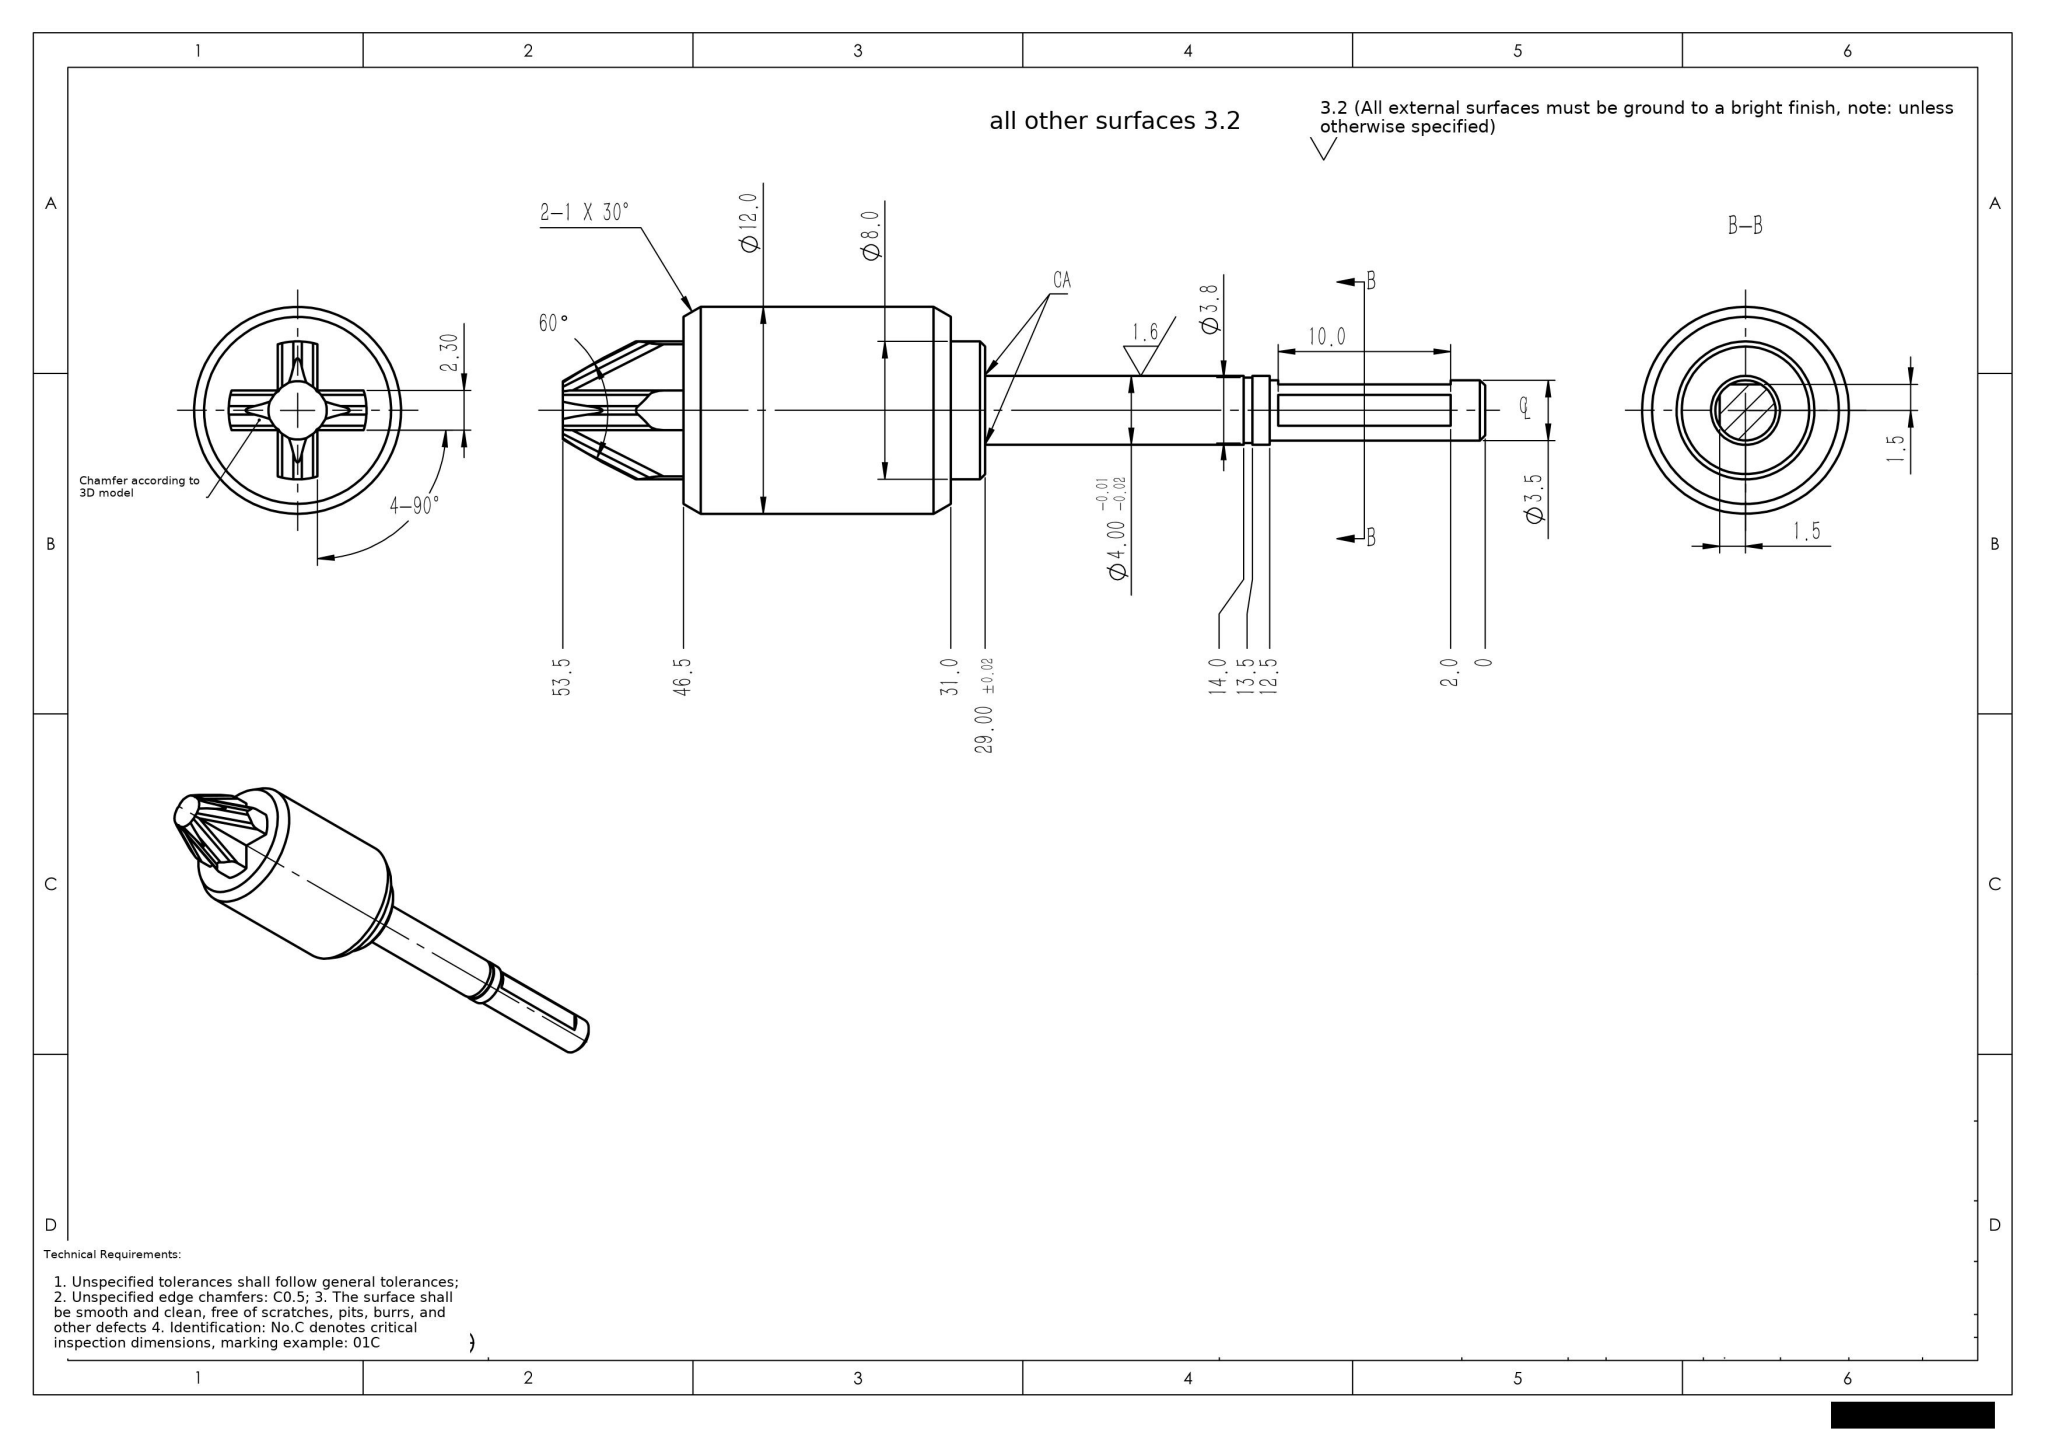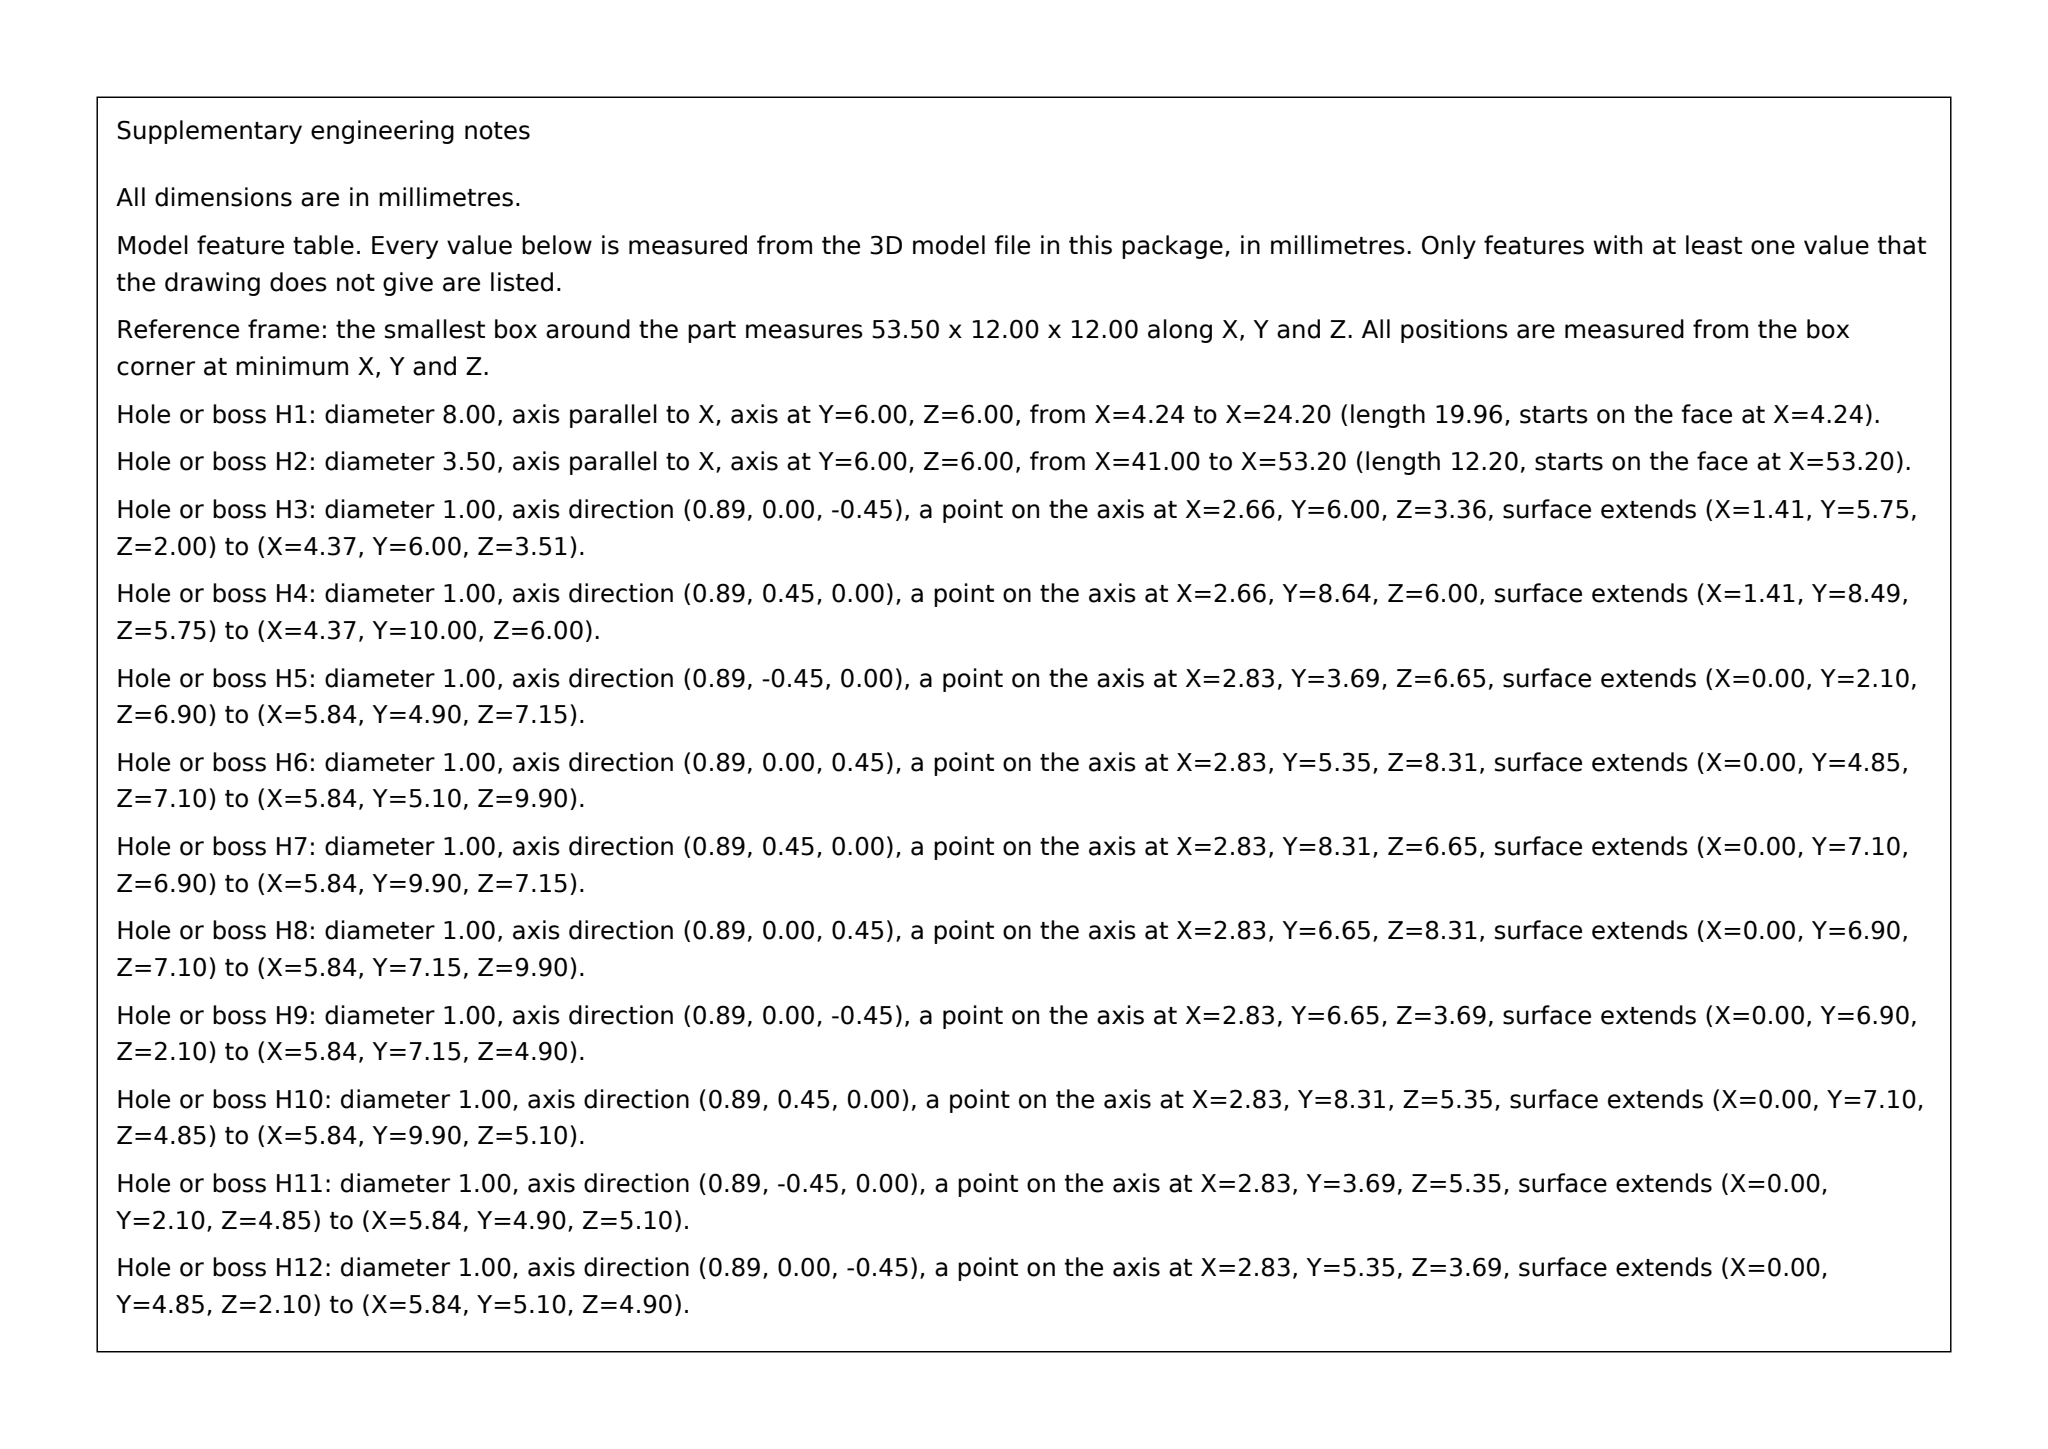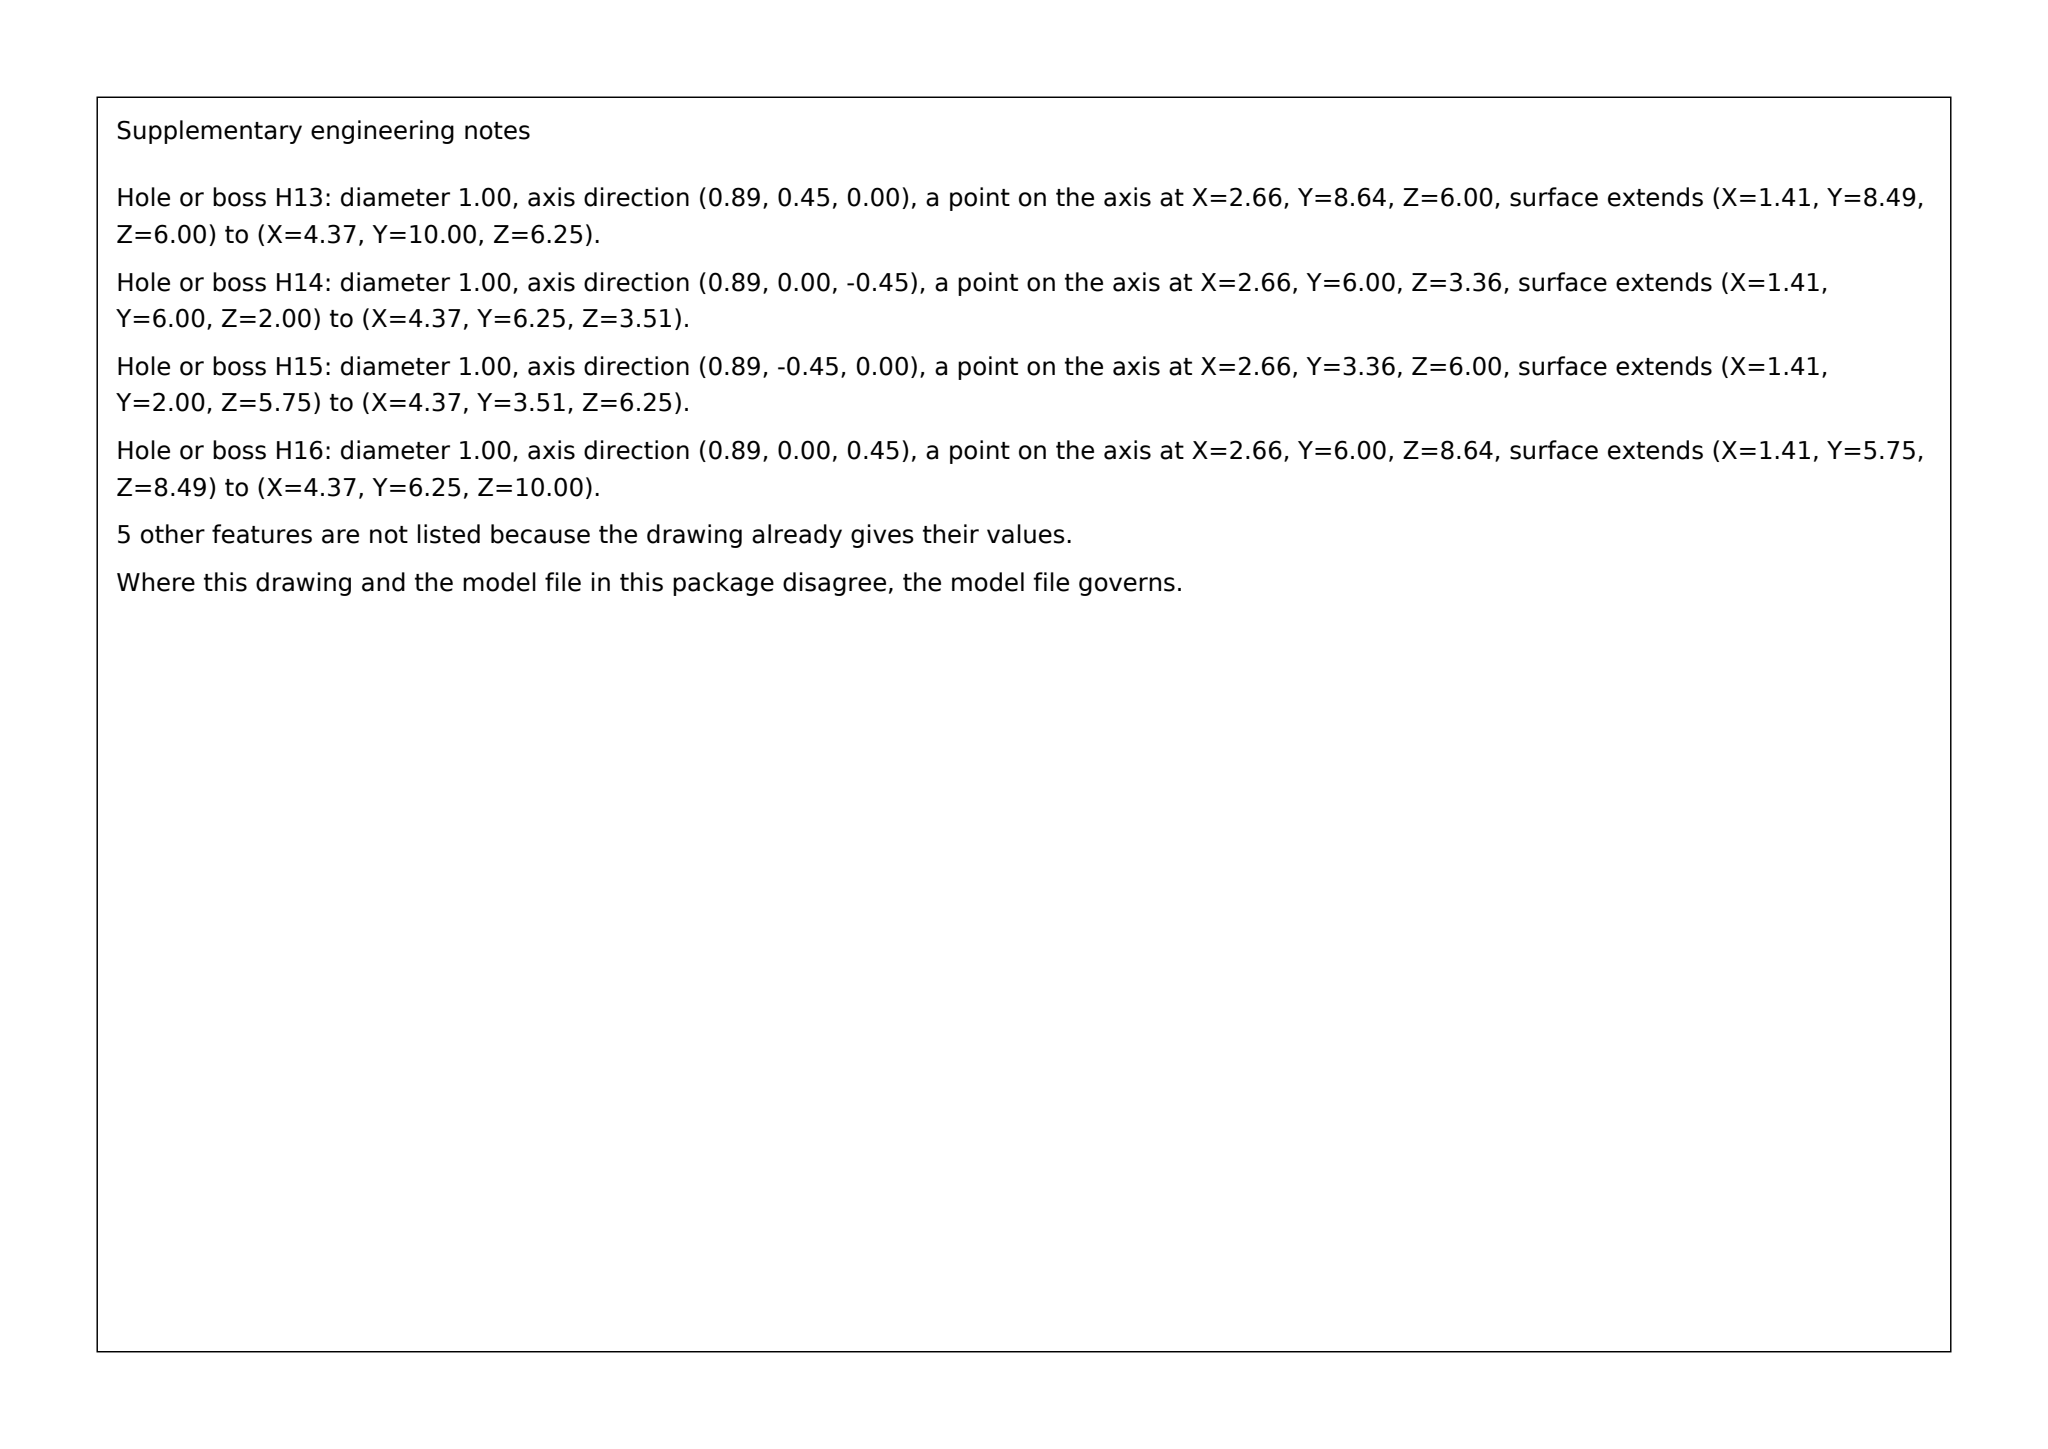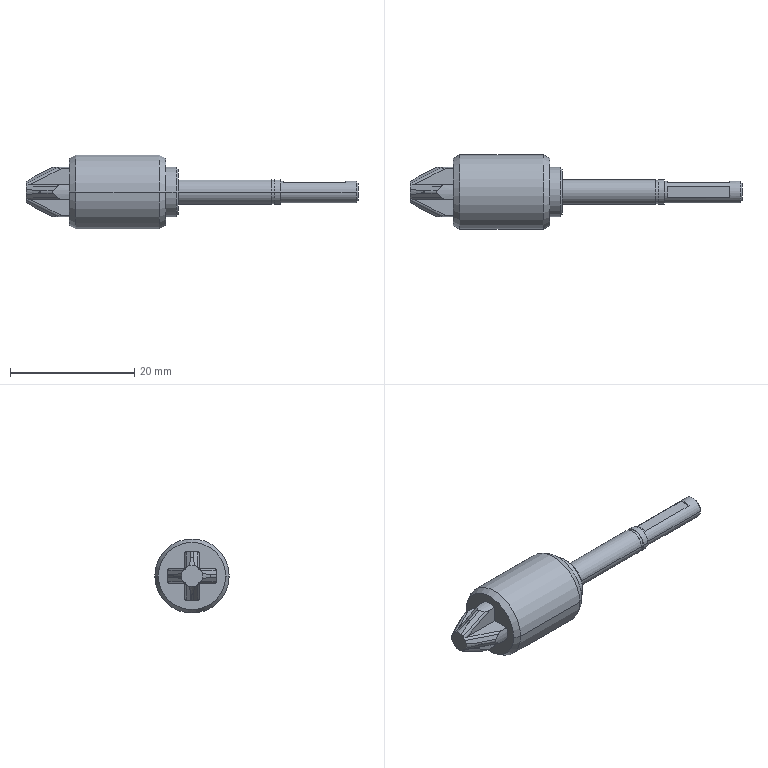Part | SolidWorks | mm | 1 solid | 74 faces | box 53.5 x 12 x 12 mm | volume 2316 mm3 | cylinder 31 | plane 30 | cone 13 | commonest cylinder face diameters 1 x14 8 x7 4 x4 3.8 x2 3.5 x2 12 x2